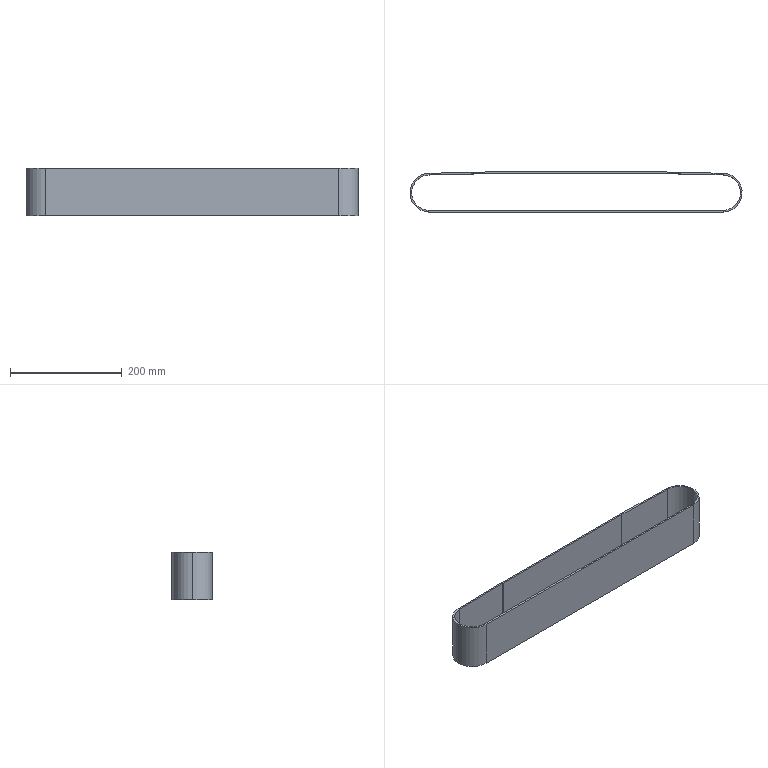Component | SolidWorks | SupportWheelAssembly-1_-SynchronousBeltLength1260-1 | 1 solid | 20 faces | box 594.5 x 72 x 85 mm | volume 321038 mm3 | cylinder 10 | plane 10 | commonest cylinder face diameters 63.5 x5 69.5 x5
build123d program:
from build123d import *

# Parameters (mm, degrees)
BOSS_EXTRUDE1_DEPTH = 42.5


with BuildPart() as part:
    # Sketch1 → Boss-Extrude1 (new, symmetric)
    with BuildSketch(Plane.XY):
        with BuildLine():
            Line((525, 34.75), (0, 34.75))
            ThreePointArc((0, 34.75), (-34.748, 0.386), (-0.772, -34.741))
            Line((-0.772, -34.741), (111.728, -37.241))
            ThreePointArc((111.728, -37.241), (112.114, -37.248), (112.5, -37.25))
            Line((112.5, -37.25), (412.5, -37.25))
            ThreePointArc((412.5, -37.25), (412.886, -37.248), (413.272, -37.241))
            Line((413.272, -37.241), (525.772, -34.741))
            ThreePointArc((525.772, -34.741), (559.748, 0.386), (525, 34.75))
        make_face()
        with BuildLine():
            Line((525, 31.75), (0, 31.75))
            ThreePointArc((0, 31.75), (-31.748, 0.3527), (-0.7054, -31.742))
            Line((-0.7054, -31.742), (111.795, -34.242))
            ThreePointArc((111.795, -34.242), (112.147, -34.248), (112.5, -34.25))
            Line((112.5, -34.25), (412.5, -34.25))
            ThreePointArc((412.5, -34.25), (412.853, -34.248), (413.205, -34.242))
            Line((413.205, -34.242), (525.705, -31.742))
            ThreePointArc((525.705, -31.742), (556.748, 0.3527), (525, 31.75))
        make_face(mode=Mode.SUBTRACT)
    extrude(amount=BOSS_EXTRUDE1_DEPTH, both=True)


solid = part.part

# Placed as in the assembly
solid = solid.moved(Location((-299.507, -197.911, 567.5), (180, 0, 0)))
STEP:
#1=COLOUR_RGB('',0.7922,0.8196,0.9333);
#2=FILL_AREA_STYLE_COLOUR('',#1);
#3=FILL_AREA_STYLE('',(#2));
#4=SURFACE_STYLE_FILL_AREA(#3);
#5=SURFACE_SIDE_STYLE('',(#4));
#6=SURFACE_STYLE_USAGE(.BOTH.,#5);
#7=PRESENTATION_STYLE_ASSIGNMENT((#6));
#8=CARTESIAN_POINT('',(-11.792,-9.042,20.669));
#9=VERTEX_POINT('',#8);
#10=CARTESIAN_POINT('',(-13.042,-7.792,20.669));
#11=VERTEX_POINT('',#10);
#12=CARTESIAN_POINT('',(-11.792,-7.792,20.669));
#13=DIRECTION('',(0.,0.,-1.));
#14=DIRECTION('',(1.,0.,0.));
#15=AXIS2_PLACEMENT_3D('',#12,#13,#14);
#16=CIRCLE('',#15,1.25);
#17=EDGE_CURVE('',#9,#11,#16,.T.);
#18=ORIENTED_EDGE('',*,*,#17,.T.);
#19=CARTESIAN_POINT('',(-13.042,-7.792,24.016));
#20=VERTEX_POINT('',#19);
#21=CARTESIAN_POINT('',(-13.042,-7.792,20.669));
#22=DIRECTION('',(0.,0.,1.));
#23=VECTOR('',#22,39.37);
#24=LINE('',#21,#23);
#25=EDGE_CURVE('',#11,#20,#24,.T.);
#26=ORIENTED_EDGE('',*,*,#25,.T.);
#27=CARTESIAN_POINT('',(-11.792,-9.042,24.016));
#28=VERTEX_POINT('',#27);
#29=CARTESIAN_POINT('',(-11.792,-7.792,24.016));
#30=DIRECTION('',(0.,0.,-1.));
#31=DIRECTION('',(1.,0.,0.));
#32=AXIS2_PLACEMENT_3D('',#29,#30,#31);
#33=CIRCLE('',#32,1.25);
#34=EDGE_CURVE('',#28,#20,#33,.T.);
#35=ORIENTED_EDGE('',*,*,#34,.F.);
#36=CARTESIAN_POINT('',(-11.792,-9.042,20.669));
#37=DIRECTION('',(0.,0.,1.));
#38=VECTOR('',#37,39.37);
#39=LINE('',#36,#38);
#40=EDGE_CURVE('',#9,#28,#39,.T.);
#41=ORIENTED_EDGE('',*,*,#40,.F.);
#42=EDGE_LOOP('',(#18,#26,#35,#41));
#43=FACE_OUTER_BOUND('',#42,.T.);
#44=CARTESIAN_POINT('',(-11.792,-7.792,20.669));
#45=DIRECTION('',(0.,0.,1.));
#46=DIRECTION('',(-1.,0.,0.));
#47=AXIS2_PLACEMENT_3D('',#44,#45,#46);
#48=CYLINDRICAL_SURFACE('',#47,1.25);
#49=ADVANCED_FACE('',(#43),#48,.F.);
#50=CARTESIAN_POINT('',(-13.16,-7.792,20.669));
#51=VERTEX_POINT('',#50);
#52=CARTESIAN_POINT('',(-11.822,-6.424,20.669));
#53=VERTEX_POINT('',#52);
#54=CARTESIAN_POINT('',(-11.792,-7.792,20.669));
#55=DIRECTION('',(0.,0.,-1.));
#56=DIRECTION('',(1.,0.,0.));
#57=AXIS2_PLACEMENT_3D('',#54,#55,#56);
#58=CIRCLE('',#57,1.368);
#59=EDGE_CURVE('',#51,#53,#58,.T.);
#60=ORIENTED_EDGE('',*,*,#59,.F.);
#61=CARTESIAN_POINT('',(-13.16,-7.792,24.016));
#62=VERTEX_POINT('',#61);
#63=CARTESIAN_POINT('',(-13.16,-7.792,20.669));
#64=DIRECTION('',(0.,0.,1.));
#65=VECTOR('',#64,39.37);
#66=LINE('',#63,#65);
#67=EDGE_CURVE('',#51,#62,#66,.T.);
#68=ORIENTED_EDGE('',*,*,#67,.T.);
#69=CARTESIAN_POINT('',(-11.822,-6.424,24.016));
#70=VERTEX_POINT('',#69);
#71=CARTESIAN_POINT('',(-11.792,-7.792,24.016));
#72=DIRECTION('',(0.,0.,-1.));
#73=DIRECTION('',(1.,0.,0.));
#74=AXIS2_PLACEMENT_3D('',#71,#72,#73);
#75=CIRCLE('',#74,1.368);
#76=EDGE_CURVE('',#62,#70,#75,.T.);
#77=ORIENTED_EDGE('',*,*,#76,.T.);
#78=CARTESIAN_POINT('',(-11.822,-6.424,20.669));
#79=DIRECTION('',(0.,0.,1.));
#80=VECTOR('',#79,39.37);
#81=LINE('',#78,#80);
#82=EDGE_CURVE('',#53,#70,#81,.T.);
#83=ORIENTED_EDGE('',*,*,#82,.F.);
#84=EDGE_LOOP('',(#60,#68,#77,#83));
#85=FACE_OUTER_BOUND('',#84,.T.);
#86=CARTESIAN_POINT('',(-11.792,-7.792,20.669));
#87=DIRECTION('',(0.,0.,1.));
#88=DIRECTION('',(-1.,0.,0.));
#89=AXIS2_PLACEMENT_3D('',#86,#87,#88);
#90=CYLINDRICAL_SURFACE('',#89,1.368);
#91=ADVANCED_FACE('',(#85),#90,.T.);
#92=CARTESIAN_POINT('',(8.908,-6.424,20.669));
#93=VERTEX_POINT('',#92);
#94=CARTESIAN_POINT('',(8.878,-9.16,20.669));
#95=VERTEX_POINT('',#94);
#96=CARTESIAN_POINT('',(8.878,-7.792,20.669));
#97=DIRECTION('',(0.,0.,-1.));
#98=DIRECTION('',(1.,0.,0.));
#99=AXIS2_PLACEMENT_3D('',#96,#97,#98);
#100=CIRCLE('',#99,1.368);
#101=EDGE_CURVE('',#93,#95,#100,.T.);
#102=ORIENTED_EDGE('',*,*,#101,.T.);
#103=CARTESIAN_POINT('',(-11.792,-9.16,20.669));
#104=VERTEX_POINT('',#103);
#105=CARTESIAN_POINT('',(8.878,-9.16,20.669));
#106=DIRECTION('',(-1.,0.,0.));
#107=VECTOR('',#106,39.37);
#108=LINE('',#105,#107);
#109=EDGE_CURVE('',#95,#104,#108,.T.);
#110=ORIENTED_EDGE('',*,*,#109,.T.);
#111=CARTESIAN_POINT('',(-11.792,-7.792,20.669));
#112=DIRECTION('',(0.,0.,-1.));
#113=DIRECTION('',(1.,0.,0.));
#114=AXIS2_PLACEMENT_3D('',#111,#112,#113);
#115=CIRCLE('',#114,1.368);
#116=EDGE_CURVE('',#104,#51,#115,.T.);
#117=ORIENTED_EDGE('',*,*,#116,.T.);
#118=ORIENTED_EDGE('',*,*,#59,.T.);
#119=CARTESIAN_POINT('',(-7.393,-6.326,20.669));
#120=VERTEX_POINT('',#119);
#121=CARTESIAN_POINT('',(-11.822,-6.424,20.669));
#122=DIRECTION('',(0.9998,0.02222,0.));
#123=VECTOR('',#122,39.37);
#124=LINE('',#121,#123);
#125=EDGE_CURVE('',#53,#120,#124,.T.);
#126=ORIENTED_EDGE('',*,*,#125,.T.);
#127=CARTESIAN_POINT('',(-7.362,-6.325,20.669));
#128=VERTEX_POINT('',#127);
#129=CARTESIAN_POINT('',(-7.362,-7.693,20.669));
#130=DIRECTION('',(0.,0.,-1.));
#131=DIRECTION('',(1.,0.,0.));
#132=AXIS2_PLACEMENT_3D('',#129,#130,#131);
#133=CIRCLE('',#132,1.368);
#134=EDGE_CURVE('',#120,#128,#133,.T.);
#135=ORIENTED_EDGE('',*,*,#134,.T.);
#136=CARTESIAN_POINT('',(4.449,-6.325,20.669));
#137=VERTEX_POINT('',#136);
#138=CARTESIAN_POINT('',(-7.362,-6.325,20.669));
#139=DIRECTION('',(1.,0.,0.));
#140=VECTOR('',#139,39.37);
#141=LINE('',#138,#140);
#142=EDGE_CURVE('',#128,#137,#141,.T.);
#143=ORIENTED_EDGE('',*,*,#142,.T.);
#144=CARTESIAN_POINT('',(4.479,-6.326,20.669));
#145=VERTEX_POINT('',#144);
#146=CARTESIAN_POINT('',(4.449,-7.693,20.669));
#147=DIRECTION('',(0.,0.,-1.));
#148=DIRECTION('',(1.,0.,0.));
#149=AXIS2_PLACEMENT_3D('',#146,#147,#148);
#150=CIRCLE('',#149,1.368);
#151=EDGE_CURVE('',#137,#145,#150,.T.);
#152=ORIENTED_EDGE('',*,*,#151,.T.);
#153=CARTESIAN_POINT('',(4.479,-6.326,20.669));
#154=DIRECTION('',(0.9998,-0.02222,0.));
#155=VECTOR('',#154,39.37);
#156=LINE('',#153,#155);
#157=EDGE_CURVE('',#145,#93,#156,.T.);
#158=ORIENTED_EDGE('',*,*,#157,.T.);
#159=EDGE_LOOP('',(#102,#110,#117,#118,#126,#135,#143,#152,#158));
#160=FACE_OUTER_BOUND('',#159,.T.);
#161=CARTESIAN_POINT('',(8.878,-9.042,20.669));
#162=VERTEX_POINT('',#161);
#163=CARTESIAN_POINT('',(8.878,-9.042,20.669));
#164=DIRECTION('',(-1.,0.,0.));
#165=VECTOR('',#164,39.37);
#166=LINE('',#163,#165);
#167=EDGE_CURVE('',#162,#9,#166,.T.);
#168=ORIENTED_EDGE('',*,*,#167,.F.);
#169=CARTESIAN_POINT('',(8.905,-6.542,20.669));
#170=VERTEX_POINT('',#169);
#171=CARTESIAN_POINT('',(8.878,-7.792,20.669));
#172=DIRECTION('',(0.,0.,-1.));
#173=DIRECTION('',(1.,0.,0.));
#174=AXIS2_PLACEMENT_3D('',#171,#172,#173);
#175=CIRCLE('',#174,1.25);
#176=EDGE_CURVE('',#170,#162,#175,.T.);
#177=ORIENTED_EDGE('',*,*,#176,.F.);
#178=CARTESIAN_POINT('',(4.476,-6.444,20.669));
#179=VERTEX_POINT('',#178);
#180=CARTESIAN_POINT('',(4.476,-6.444,20.669));
#181=DIRECTION('',(0.9998,-0.02222,0.));
#182=VECTOR('',#181,39.37);
#183=LINE('',#180,#182);
#184=EDGE_CURVE('',#179,#170,#183,.T.);
#185=ORIENTED_EDGE('',*,*,#184,.F.);
#186=CARTESIAN_POINT('',(4.449,-6.443,20.669));
#187=VERTEX_POINT('',#186);
#188=CARTESIAN_POINT('',(4.449,-7.693,20.669));
#189=DIRECTION('',(0.,0.,-1.));
#190=DIRECTION('',(1.,0.,0.));
#191=AXIS2_PLACEMENT_3D('',#188,#189,#190);
#192=CIRCLE('',#191,1.25);
#193=EDGE_CURVE('',#187,#179,#192,.T.);
#194=ORIENTED_EDGE('',*,*,#193,.F.);
#195=CARTESIAN_POINT('',(-7.362,-6.443,20.669));
#196=VERTEX_POINT('',#195);
#197=CARTESIAN_POINT('',(-7.362,-6.443,20.669));
#198=DIRECTION('',(1.,0.,0.));
#199=VECTOR('',#198,39.37);
#200=LINE('',#197,#199);
#201=EDGE_CURVE('',#196,#187,#200,.T.);
#202=ORIENTED_EDGE('',*,*,#201,.F.);
#203=CARTESIAN_POINT('',(-7.39,-6.444,20.669));
#204=VERTEX_POINT('',#203);
#205=CARTESIAN_POINT('',(-7.362,-7.693,20.669));
#206=DIRECTION('',(0.,0.,-1.));
#207=DIRECTION('',(1.,0.,0.));
#208=AXIS2_PLACEMENT_3D('',#205,#206,#207);
#209=CIRCLE('',#208,1.25);
#210=EDGE_CURVE('',#204,#196,#209,.T.);
#211=ORIENTED_EDGE('',*,*,#210,.F.);
#212=CARTESIAN_POINT('',(-11.819,-6.542,20.669));
#213=VERTEX_POINT('',#212);
#214=CARTESIAN_POINT('',(-11.819,-6.542,20.669));
#215=DIRECTION('',(0.9998,0.02222,0.));
#216=VECTOR('',#215,39.37);
#217=LINE('',#214,#216);
#218=EDGE_CURVE('',#213,#204,#217,.T.);
#219=ORIENTED_EDGE('',*,*,#218,.F.);
#220=CARTESIAN_POINT('',(-11.792,-7.792,20.669));
#221=DIRECTION('',(0.,0.,-1.));
#222=DIRECTION('',(1.,0.,0.));
#223=AXIS2_PLACEMENT_3D('',#220,#221,#222);
#224=CIRCLE('',#223,1.25);
#225=EDGE_CURVE('',#11,#213,#224,.T.);
#226=ORIENTED_EDGE('',*,*,#225,.F.);
#227=ORIENTED_EDGE('',*,*,#17,.F.);
#228=EDGE_LOOP('',(#168,#177,#185,#194,#202,#211,#219,#226,#227));
#229=FACE_BOUND('',#228,.T.);
#230=CARTESIAN_POINT('',(8.878,-7.792,20.669));
#231=DIRECTION('',(0.,0.,-1.));
#232=DIRECTION('',(1.,0.,0.));
#233=AXIS2_PLACEMENT_3D('',#230,#231,#232);
#234=PLANE('',#233);
#235=ADVANCED_FACE('',(#160,#229),#234,.T.);
#236=CARTESIAN_POINT('',(8.908,-6.424,24.016));
#237=VERTEX_POINT('',#236);
#238=CARTESIAN_POINT('',(8.878,-9.16,24.016));
#239=VERTEX_POINT('',#238);
#240=CARTESIAN_POINT('',(8.878,-7.792,24.016));
#241=DIRECTION('',(0.,0.,-1.));
#242=DIRECTION('',(1.,0.,0.));
#243=AXIS2_PLACEMENT_3D('',#240,#241,#242);
#244=CIRCLE('',#243,1.368);
#245=EDGE_CURVE('',#237,#239,#244,.T.);
#246=ORIENTED_EDGE('',*,*,#245,.F.);
#247=CARTESIAN_POINT('',(4.479,-6.326,24.016));
#248=VERTEX_POINT('',#247);
#249=CARTESIAN_POINT('',(4.479,-6.326,24.016));
#250=DIRECTION('',(0.9998,-0.02222,0.));
#251=VECTOR('',#250,39.37);
#252=LINE('',#249,#251);
#253=EDGE_CURVE('',#248,#237,#252,.T.);
#254=ORIENTED_EDGE('',*,*,#253,.F.);
#255=CARTESIAN_POINT('',(4.449,-6.325,24.016));
#256=VERTEX_POINT('',#255);
#257=CARTESIAN_POINT('',(4.449,-7.693,24.016));
#258=DIRECTION('',(0.,0.,-1.));
#259=DIRECTION('',(1.,0.,0.));
#260=AXIS2_PLACEMENT_3D('',#257,#258,#259);
#261=CIRCLE('',#260,1.368);
#262=EDGE_CURVE('',#256,#248,#261,.T.);
#263=ORIENTED_EDGE('',*,*,#262,.F.);
#264=CARTESIAN_POINT('',(-7.362,-6.325,24.016));
#265=VERTEX_POINT('',#264);
#266=CARTESIAN_POINT('',(-7.362,-6.325,24.016));
#267=DIRECTION('',(1.,0.,0.));
#268=VECTOR('',#267,39.37);
#269=LINE('',#266,#268);
#270=EDGE_CURVE('',#265,#256,#269,.T.);
#271=ORIENTED_EDGE('',*,*,#270,.F.);
#272=CARTESIAN_POINT('',(-7.393,-6.326,24.016));
#273=VERTEX_POINT('',#272);
#274=CARTESIAN_POINT('',(-7.362,-7.693,24.016));
#275=DIRECTION('',(0.,0.,-1.));
#276=DIRECTION('',(1.,0.,0.));
#277=AXIS2_PLACEMENT_3D('',#274,#275,#276);
#278=CIRCLE('',#277,1.368);
#279=EDGE_CURVE('',#273,#265,#278,.T.);
#280=ORIENTED_EDGE('',*,*,#279,.F.);
#281=CARTESIAN_POINT('',(-11.822,-6.424,24.016));
#282=DIRECTION('',(0.9998,0.02222,0.));
#283=VECTOR('',#282,39.37);
#284=LINE('',#281,#283);
#285=EDGE_CURVE('',#70,#273,#284,.T.);
#286=ORIENTED_EDGE('',*,*,#285,.F.);
#287=ORIENTED_EDGE('',*,*,#76,.F.);
#288=CARTESIAN_POINT('',(-11.792,-9.16,24.016));
#289=VERTEX_POINT('',#288);
#290=CARTESIAN_POINT('',(-11.792,-7.792,24.016));
#291=DIRECTION('',(0.,0.,-1.));
#292=DIRECTION('',(1.,0.,0.));
#293=AXIS2_PLACEMENT_3D('',#290,#291,#292);
#294=CIRCLE('',#293,1.368);
#295=EDGE_CURVE('',#289,#62,#294,.T.);
#296=ORIENTED_EDGE('',*,*,#295,.F.);
#297=CARTESIAN_POINT('',(8.878,-9.16,24.016));
#298=DIRECTION('',(-1.,0.,0.));
#299=VECTOR('',#298,39.37);
#300=LINE('',#297,#299);
#301=EDGE_CURVE('',#239,#289,#300,.T.);
#302=ORIENTED_EDGE('',*,*,#301,.F.);
#303=EDGE_LOOP('',(#246,#254,#263,#271,#280,#286,#287,#296,#302));
#304=FACE_OUTER_BOUND('',#303,.T.);
#305=CARTESIAN_POINT('',(8.905,-6.542,24.016));
#306=VERTEX_POINT('',#305);
#307=CARTESIAN_POINT('',(8.878,-9.042,24.016));
#308=VERTEX_POINT('',#307);
#309=CARTESIAN_POINT('',(8.878,-7.792,24.016));
#310=DIRECTION('',(0.,0.,-1.));
#311=DIRECTION('',(1.,0.,0.));
#312=AXIS2_PLACEMENT_3D('',#309,#310,#311);
#313=CIRCLE('',#312,1.25);
#314=EDGE_CURVE('',#306,#308,#313,.T.);
#315=ORIENTED_EDGE('',*,*,#314,.T.);
#316=CARTESIAN_POINT('',(8.878,-9.042,24.016));
#317=DIRECTION('',(-1.,0.,0.));
#318=VECTOR('',#317,39.37);
#319=LINE('',#316,#318);
#320=EDGE_CURVE('',#308,#28,#319,.T.);
#321=ORIENTED_EDGE('',*,*,#320,.T.);
#322=ORIENTED_EDGE('',*,*,#34,.T.);
#323=CARTESIAN_POINT('',(-11.819,-6.542,24.016));
#324=VERTEX_POINT('',#323);
#325=CARTESIAN_POINT('',(-11.792,-7.792,24.016));
#326=DIRECTION('',(0.,0.,-1.));
#327=DIRECTION('',(1.,0.,0.));
#328=AXIS2_PLACEMENT_3D('',#325,#326,#327);
#329=CIRCLE('',#328,1.25);
#330=EDGE_CURVE('',#20,#324,#329,.T.);
#331=ORIENTED_EDGE('',*,*,#330,.T.);
#332=CARTESIAN_POINT('',(-7.39,-6.444,24.016));
#333=VERTEX_POINT('',#332);
#334=CARTESIAN_POINT('',(-11.819,-6.542,24.016));
#335=DIRECTION('',(0.9998,0.02222,0.));
#336=VECTOR('',#335,39.37);
#337=LINE('',#334,#336);
#338=EDGE_CURVE('',#324,#333,#337,.T.);
#339=ORIENTED_EDGE('',*,*,#338,.T.);
#340=CARTESIAN_POINT('',(-7.362,-6.443,24.016));
#341=VERTEX_POINT('',#340);
#342=CARTESIAN_POINT('',(-7.362,-7.693,24.016));
#343=DIRECTION('',(0.,0.,-1.));
#344=DIRECTION('',(1.,0.,0.));
#345=AXIS2_PLACEMENT_3D('',#342,#343,#344);
#346=CIRCLE('',#345,1.25);
#347=EDGE_CURVE('',#333,#341,#346,.T.);
#348=ORIENTED_EDGE('',*,*,#347,.T.);
#349=CARTESIAN_POINT('',(4.449,-6.443,24.016));
#350=VERTEX_POINT('',#349);
#351=CARTESIAN_POINT('',(-7.362,-6.443,24.016));
#352=DIRECTION('',(1.,0.,0.));
#353=VECTOR('',#352,39.37);
#354=LINE('',#351,#353);
#355=EDGE_CURVE('',#341,#350,#354,.T.);
#356=ORIENTED_EDGE('',*,*,#355,.T.);
#357=CARTESIAN_POINT('',(4.476,-6.444,24.016));
#358=VERTEX_POINT('',#357);
#359=CARTESIAN_POINT('',(4.449,-7.693,24.016));
#360=DIRECTION('',(0.,0.,-1.));
#361=DIRECTION('',(1.,0.,0.));
#362=AXIS2_PLACEMENT_3D('',#359,#360,#361);
#363=CIRCLE('',#362,1.25);
#364=EDGE_CURVE('',#350,#358,#363,.T.);
#365=ORIENTED_EDGE('',*,*,#364,.T.);
#366=CARTESIAN_POINT('',(4.476,-6.444,24.016));
#367=DIRECTION('',(0.9998,-0.02222,0.));
#368=VECTOR('',#367,39.37);
#369=LINE('',#366,#368);
#370=EDGE_CURVE('',#358,#306,#369,.T.);
#371=ORIENTED_EDGE('',*,*,#370,.T.);
#372=EDGE_LOOP('',(#315,#321,#322,#331,#339,#348,#356,#365,#371));
#373=FACE_BOUND('',#372,.T.);
#374=CARTESIAN_POINT('',(8.878,-7.792,24.016));
#375=DIRECTION('',(0.,0.,-1.));
#376=DIRECTION('',(1.,0.,0.));
#377=AXIS2_PLACEMENT_3D('',#374,#375,#376);
#378=PLANE('',#377);
#379=ADVANCED_FACE('',(#304,#373),#378,.F.);
#380=ORIENTED_EDGE('',*,*,#245,.T.);
#381=CARTESIAN_POINT('',(8.878,-9.16,20.669));
#382=DIRECTION('',(0.,0.,1.));
#383=VECTOR('',#382,39.37);
#384=LINE('',#381,#383);
#385=EDGE_CURVE('',#95,#239,#384,.T.);
#386=ORIENTED_EDGE('',*,*,#385,.F.);
#387=ORIENTED_EDGE('',*,*,#101,.F.);
#388=CARTESIAN_POINT('',(8.908,-6.424,20.669));
#389=DIRECTION('',(0.,0.,1.));
#390=VECTOR('',#389,39.37);
#391=LINE('',#388,#390);
#392=EDGE_CURVE('',#93,#237,#391,.T.);
#393=ORIENTED_EDGE('',*,*,#392,.T.);
#394=EDGE_LOOP('',(#380,#386,#387,#393));
#395=FACE_OUTER_BOUND('',#394,.T.);
#396=CARTESIAN_POINT('',(8.878,-7.792,20.669));
#397=DIRECTION('',(0.,0.,1.));
#398=DIRECTION('',(-1.,0.,0.));
#399=AXIS2_PLACEMENT_3D('',#396,#397,#398);
#400=CYLINDRICAL_SURFACE('',#399,1.368);
#401=ADVANCED_FACE('',(#395),#400,.T.);
#402=ORIENTED_EDGE('',*,*,#301,.T.);
#403=CARTESIAN_POINT('',(-11.792,-9.16,20.669));
#404=DIRECTION('',(0.,0.,1.));
#405=VECTOR('',#404,39.37);
#406=LINE('',#403,#405);
#407=EDGE_CURVE('',#104,#289,#406,.T.);
#408=ORIENTED_EDGE('',*,*,#407,.F.);
#409=ORIENTED_EDGE('',*,*,#109,.F.);
#410=ORIENTED_EDGE('',*,*,#385,.T.);
#411=EDGE_LOOP('',(#402,#408,#409,#410));
#412=FACE_OUTER_BOUND('',#411,.T.);
#413=CARTESIAN_POINT('',(8.878,-9.16,20.669));
#414=DIRECTION('',(0.,1.,0.));
#415=DIRECTION('',(0.,0.,1.));
#416=AXIS2_PLACEMENT_3D('',#413,#414,#415);
#417=PLANE('',#416);
#418=ADVANCED_FACE('',(#412),#417,.F.);
#419=ORIENTED_EDGE('',*,*,#67,.F.);
#420=ORIENTED_EDGE('',*,*,#116,.F.);
#421=ORIENTED_EDGE('',*,*,#407,.T.);
#422=ORIENTED_EDGE('',*,*,#295,.T.);
#423=EDGE_LOOP('',(#419,#420,#421,#422));
#424=FACE_OUTER_BOUND('',#423,.T.);
#425=CARTESIAN_POINT('',(-11.792,-7.792,20.669));
#426=DIRECTION('',(0.,0.,1.));
#427=DIRECTION('',(-1.,0.,0.));
#428=AXIS2_PLACEMENT_3D('',#425,#426,#427);
#429=CYLINDRICAL_SURFACE('',#428,1.368);
#430=ADVANCED_FACE('',(#424),#429,.T.);
#431=ORIENTED_EDGE('',*,*,#285,.T.);
#432=CARTESIAN_POINT('',(-7.393,-6.326,20.669));
#433=DIRECTION('',(0.,0.,1.));
#434=VECTOR('',#433,39.37);
#435=LINE('',#432,#434);
#436=EDGE_CURVE('',#120,#273,#435,.T.);
#437=ORIENTED_EDGE('',*,*,#436,.F.);
#438=ORIENTED_EDGE('',*,*,#125,.F.);
#439=ORIENTED_EDGE('',*,*,#82,.T.);
#440=EDGE_LOOP('',(#431,#437,#438,#439));
#441=FACE_OUTER_BOUND('',#440,.T.);
#442=CARTESIAN_POINT('',(-11.822,-6.424,20.669));
#443=DIRECTION('',(0.02222,-0.9998,0.));
#444=DIRECTION('',(-0.9998,-0.02222,0.));
#445=AXIS2_PLACEMENT_3D('',#442,#443,#444);
#446=PLANE('',#445);
#447=ADVANCED_FACE('',(#441),#446,.F.);
#448=ORIENTED_EDGE('',*,*,#279,.T.);
#449=CARTESIAN_POINT('',(-7.362,-6.325,20.669));
#450=DIRECTION('',(0.,0.,1.));
#451=VECTOR('',#450,39.37);
#452=LINE('',#449,#451);
#453=EDGE_CURVE('',#128,#265,#452,.T.);
#454=ORIENTED_EDGE('',*,*,#453,.F.);
#455=ORIENTED_EDGE('',*,*,#134,.F.);
#456=ORIENTED_EDGE('',*,*,#436,.T.);
#457=EDGE_LOOP('',(#448,#454,#455,#456));
#458=FACE_OUTER_BOUND('',#457,.T.);
#459=CARTESIAN_POINT('',(-7.362,-7.693,20.669));
#460=DIRECTION('',(0.,0.,1.));
#461=DIRECTION('',(-1.,0.,0.));
#462=AXIS2_PLACEMENT_3D('',#459,#460,#461);
#463=CYLINDRICAL_SURFACE('',#462,1.368);
#464=ADVANCED_FACE('',(#458),#463,.T.);
#465=ORIENTED_EDGE('',*,*,#270,.T.);
#466=CARTESIAN_POINT('',(4.449,-6.325,20.669));
#467=DIRECTION('',(0.,0.,1.));
#468=VECTOR('',#467,39.37);
#469=LINE('',#466,#468);
#470=EDGE_CURVE('',#137,#256,#469,.T.);
#471=ORIENTED_EDGE('',*,*,#470,.F.);
#472=ORIENTED_EDGE('',*,*,#142,.F.);
#473=ORIENTED_EDGE('',*,*,#453,.T.);
#474=EDGE_LOOP('',(#465,#471,#472,#473));
#475=FACE_OUTER_BOUND('',#474,.T.);
#476=CARTESIAN_POINT('',(-7.362,-6.325,20.669));
#477=DIRECTION('',(0.,-1.,0.));
#478=DIRECTION('',(0.,0.,-1.));
#479=AXIS2_PLACEMENT_3D('',#476,#477,#478);
#480=PLANE('',#479);
#481=ADVANCED_FACE('',(#475),#480,.F.);
#482=ORIENTED_EDGE('',*,*,#262,.T.);
#483=CARTESIAN_POINT('',(4.479,-6.326,20.669));
#484=DIRECTION('',(0.,0.,1.));
#485=VECTOR('',#484,39.37);
#486=LINE('',#483,#485);
#487=EDGE_CURVE('',#145,#248,#486,.T.);
#488=ORIENTED_EDGE('',*,*,#487,.F.);
#489=ORIENTED_EDGE('',*,*,#151,.F.);
#490=ORIENTED_EDGE('',*,*,#470,.T.);
#491=EDGE_LOOP('',(#482,#488,#489,#490));
#492=FACE_OUTER_BOUND('',#491,.T.);
#493=CARTESIAN_POINT('',(4.449,-7.693,20.669));
#494=DIRECTION('',(0.,0.,1.));
#495=DIRECTION('',(-1.,0.,0.));
#496=AXIS2_PLACEMENT_3D('',#493,#494,#495);
#497=CYLINDRICAL_SURFACE('',#496,1.368);
#498=ADVANCED_FACE('',(#492),#497,.T.);
#499=ORIENTED_EDGE('',*,*,#253,.T.);
#500=ORIENTED_EDGE('',*,*,#392,.F.);
#501=ORIENTED_EDGE('',*,*,#157,.F.);
#502=ORIENTED_EDGE('',*,*,#487,.T.);
#503=EDGE_LOOP('',(#499,#500,#501,#502));
#504=FACE_OUTER_BOUND('',#503,.T.);
#505=CARTESIAN_POINT('',(4.479,-6.326,20.669));
#506=DIRECTION('',(-0.02222,-0.9998,0.));
#507=DIRECTION('',(-0.9998,0.02222,0.));
#508=AXIS2_PLACEMENT_3D('',#505,#506,#507);
#509=PLANE('',#508);
#510=ADVANCED_FACE('',(#504),#509,.F.);
#511=ORIENTED_EDGE('',*,*,#314,.F.);
#512=CARTESIAN_POINT('',(8.905,-6.542,20.669));
#513=DIRECTION('',(0.,0.,1.));
#514=VECTOR('',#513,39.37);
#515=LINE('',#512,#514);
#516=EDGE_CURVE('',#170,#306,#515,.T.);
#517=ORIENTED_EDGE('',*,*,#516,.F.);
#518=ORIENTED_EDGE('',*,*,#176,.T.);
#519=CARTESIAN_POINT('',(8.878,-9.042,20.669));
#520=DIRECTION('',(0.,0.,1.));
#521=VECTOR('',#520,39.37);
#522=LINE('',#519,#521);
#523=EDGE_CURVE('',#162,#308,#522,.T.);
#524=ORIENTED_EDGE('',*,*,#523,.T.);
#525=EDGE_LOOP('',(#511,#517,#518,#524));
#526=FACE_OUTER_BOUND('',#525,.T.);
#527=CARTESIAN_POINT('',(8.878,-7.792,20.669));
#528=DIRECTION('',(0.,0.,1.));
#529=DIRECTION('',(-1.,0.,0.));
#530=AXIS2_PLACEMENT_3D('',#527,#528,#529);
#531=CYLINDRICAL_SURFACE('',#530,1.25);
#532=ADVANCED_FACE('',(#526),#531,.F.);
#533=ORIENTED_EDGE('',*,*,#320,.F.);
#534=ORIENTED_EDGE('',*,*,#523,.F.);
#535=ORIENTED_EDGE('',*,*,#167,.T.);
#536=ORIENTED_EDGE('',*,*,#40,.T.);
#537=EDGE_LOOP('',(#533,#534,#535,#536));
#538=FACE_OUTER_BOUND('',#537,.T.);
#539=CARTESIAN_POINT('',(8.878,-9.042,20.669));
#540=DIRECTION('',(0.,1.,0.));
#541=DIRECTION('',(0.,0.,1.));
#542=AXIS2_PLACEMENT_3D('',#539,#540,#541);
#543=PLANE('',#542);
#544=ADVANCED_FACE('',(#538),#543,.T.);
#545=ORIENTED_EDGE('',*,*,#25,.F.);
#546=ORIENTED_EDGE('',*,*,#225,.T.);
#547=CARTESIAN_POINT('',(-11.819,-6.542,20.669));
#548=DIRECTION('',(0.,0.,1.));
#549=VECTOR('',#548,39.37);
#550=LINE('',#547,#549);
#551=EDGE_CURVE('',#213,#324,#550,.T.);
#552=ORIENTED_EDGE('',*,*,#551,.T.);
#553=ORIENTED_EDGE('',*,*,#330,.F.);
#554=EDGE_LOOP('',(#545,#546,#552,#553));
#555=FACE_OUTER_BOUND('',#554,.T.);
#556=CARTESIAN_POINT('',(-11.792,-7.792,20.669));
#557=DIRECTION('',(0.,0.,1.));
#558=DIRECTION('',(-1.,0.,0.));
#559=AXIS2_PLACEMENT_3D('',#556,#557,#558);
#560=CYLINDRICAL_SURFACE('',#559,1.25);
#561=ADVANCED_FACE('',(#555),#560,.F.);
#562=ORIENTED_EDGE('',*,*,#338,.F.);
#563=ORIENTED_EDGE('',*,*,#551,.F.);
#564=ORIENTED_EDGE('',*,*,#218,.T.);
#565=CARTESIAN_POINT('',(-7.39,-6.444,20.669));
#566=DIRECTION('',(0.,0.,1.));
#567=VECTOR('',#566,39.37);
#568=LINE('',#565,#567);
#569=EDGE_CURVE('',#204,#333,#568,.T.);
#570=ORIENTED_EDGE('',*,*,#569,.T.);
#571=EDGE_LOOP('',(#562,#563,#564,#570));
#572=FACE_OUTER_BOUND('',#571,.T.);
#573=CARTESIAN_POINT('',(-11.819,-6.542,20.669));
#574=DIRECTION('',(0.02222,-0.9998,0.));
#575=DIRECTION('',(-0.9998,-0.02222,0.));
#576=AXIS2_PLACEMENT_3D('',#573,#574,#575);
#577=PLANE('',#576);
#578=ADVANCED_FACE('',(#572),#577,.T.);
#579=ORIENTED_EDGE('',*,*,#347,.F.);
#580=ORIENTED_EDGE('',*,*,#569,.F.);
#581=ORIENTED_EDGE('',*,*,#210,.T.);
#582=CARTESIAN_POINT('',(-7.362,-6.443,20.669));
#583=DIRECTION('',(0.,0.,1.));
#584=VECTOR('',#583,39.37);
#585=LINE('',#582,#584);
#586=EDGE_CURVE('',#196,#341,#585,.T.);
#587=ORIENTED_EDGE('',*,*,#586,.T.);
#588=EDGE_LOOP('',(#579,#580,#581,#587));
#589=FACE_OUTER_BOUND('',#588,.T.);
#590=CARTESIAN_POINT('',(-7.362,-7.693,20.669));
#591=DIRECTION('',(0.,0.,1.));
#592=DIRECTION('',(-1.,0.,0.));
#593=AXIS2_PLACEMENT_3D('',#590,#591,#592);
#594=CYLINDRICAL_SURFACE('',#593,1.25);
#595=ADVANCED_FACE('',(#589),#594,.F.);
#596=ORIENTED_EDGE('',*,*,#355,.F.);
#597=ORIENTED_EDGE('',*,*,#586,.F.);
#598=ORIENTED_EDGE('',*,*,#201,.T.);
#599=CARTESIAN_POINT('',(4.449,-6.443,20.669));
#600=DIRECTION('',(0.,0.,1.));
#601=VECTOR('',#600,39.37);
#602=LINE('',#599,#601);
#603=EDGE_CURVE('',#187,#350,#602,.T.);
#604=ORIENTED_EDGE('',*,*,#603,.T.);
#605=EDGE_LOOP('',(#596,#597,#598,#604));
#606=FACE_OUTER_BOUND('',#605,.T.);
#607=CARTESIAN_POINT('',(-7.362,-6.443,20.669));
#608=DIRECTION('',(0.,-1.,0.));
#609=DIRECTION('',(0.,0.,-1.));
#610=AXIS2_PLACEMENT_3D('',#607,#608,#609);
#611=PLANE('',#610);
#612=ADVANCED_FACE('',(#606),#611,.T.);
#613=ORIENTED_EDGE('',*,*,#364,.F.);
#614=ORIENTED_EDGE('',*,*,#603,.F.);
#615=ORIENTED_EDGE('',*,*,#193,.T.);
#616=CARTESIAN_POINT('',(4.476,-6.444,20.669));
#617=DIRECTION('',(0.,0.,1.));
#618=VECTOR('',#617,39.37);
#619=LINE('',#616,#618);
#620=EDGE_CURVE('',#179,#358,#619,.T.);
#621=ORIENTED_EDGE('',*,*,#620,.T.);
#622=EDGE_LOOP('',(#613,#614,#615,#621));
#623=FACE_OUTER_BOUND('',#622,.T.);
#624=CARTESIAN_POINT('',(4.449,-7.693,20.669));
#625=DIRECTION('',(0.,0.,1.));
#626=DIRECTION('',(-1.,0.,0.));
#627=AXIS2_PLACEMENT_3D('',#624,#625,#626);
#628=CYLINDRICAL_SURFACE('',#627,1.25);
#629=ADVANCED_FACE('',(#623),#628,.F.);
#630=ORIENTED_EDGE('',*,*,#370,.F.);
#631=ORIENTED_EDGE('',*,*,#620,.F.);
#632=ORIENTED_EDGE('',*,*,#184,.T.);
#633=ORIENTED_EDGE('',*,*,#516,.T.);
#634=EDGE_LOOP('',(#630,#631,#632,#633));
#635=FACE_OUTER_BOUND('',#634,.T.);
#636=CARTESIAN_POINT('',(4.476,-6.444,20.669));
#637=DIRECTION('',(-0.02222,-0.9998,0.));
#638=DIRECTION('',(-0.9998,0.02222,0.));
#639=AXIS2_PLACEMENT_3D('',#636,#637,#638);
#640=PLANE('',#639);
#641=ADVANCED_FACE('',(#635),#640,.T.);
#642=CLOSED_SHELL('',(#49,#91,#235,#379,#401,#418,#430,#447,#464,#481,#498,#510,#532,#544,#561,#578,#595,#612,#629,#641));
#643=MANIFOLD_SOLID_BREP('',#642);
#644=STYLED_ITEM('',(#7),#643);
#645=(LENGTH_UNIT()NAMED_UNIT(*)SI_UNIT($,.METRE.));
#646=LENGTH_MEASURE_WITH_UNIT(LENGTH_MEASURE(0.0254),#645);
#647=DIMENSIONAL_EXPONENTS(1.,0.,0.,0.,0.,0.,0.);
#648=(CONVERSION_BASED_UNIT('',#646)LENGTH_UNIT()NAMED_UNIT(#647));
#649=UNCERTAINTY_MEASURE_WITH_UNIT(LENGTH_MEASURE(0.00001),#648,'','');
#650=(NAMED_UNIT(*)PLANE_ANGLE_UNIT()SI_UNIT($,.RADIAN.));
#651=(NAMED_UNIT(*)SI_UNIT($,.STERADIAN.)SOLID_ANGLE_UNIT());
#652=(GEOMETRIC_REPRESENTATION_CONTEXT(3)GLOBAL_UNCERTAINTY_ASSIGNED_CONTEXT((#649))GLOBAL_UNIT_ASSIGNED_CONTEXT((#648,#650,#651))REPRESENTATION_CONTEXT('',''));
#653=MECHANICAL_DESIGN_GEOMETRIC_PRESENTATION_REPRESENTATION('',(#644),#652);
#654=CARTESIAN_POINT('',(0.,0.,0.));
#655=DIRECTION('',(0.,0.,1.));
#656=DIRECTION('',(1.,0.,0.));
#657=AXIS2_PLACEMENT_3D('',#654,#655,#656);
#658=(LENGTH_UNIT()NAMED_UNIT(*)SI_UNIT($,.METRE.));
#659=LENGTH_MEASURE_WITH_UNIT(LENGTH_MEASURE(0.0254),#658);
#660=DIMENSIONAL_EXPONENTS(1.,0.,0.,0.,0.,0.,0.);
#661=(CONVERSION_BASED_UNIT('',#659)LENGTH_UNIT()NAMED_UNIT(#660));
#662=UNCERTAINTY_MEASURE_WITH_UNIT(LENGTH_MEASURE(0.00001),#661,'','');
#663=(NAMED_UNIT(*)PLANE_ANGLE_UNIT()SI_UNIT($,.RADIAN.));
#664=(NAMED_UNIT(*)SI_UNIT($,.STERADIAN.)SOLID_ANGLE_UNIT());
#665=(GEOMETRIC_REPRESENTATION_CONTEXT(3)GLOBAL_UNCERTAINTY_ASSIGNED_CONTEXT((#662))GLOBAL_UNIT_ASSIGNED_CONTEXT((#661,#663,#664))REPRESENTATION_CONTEXT('',''));
#666=ADVANCED_BREP_SHAPE_REPRESENTATION('',(#643,#657),#665);
#667=PRESENTATION_LAYER_ASSIGNMENT('','',(#644));